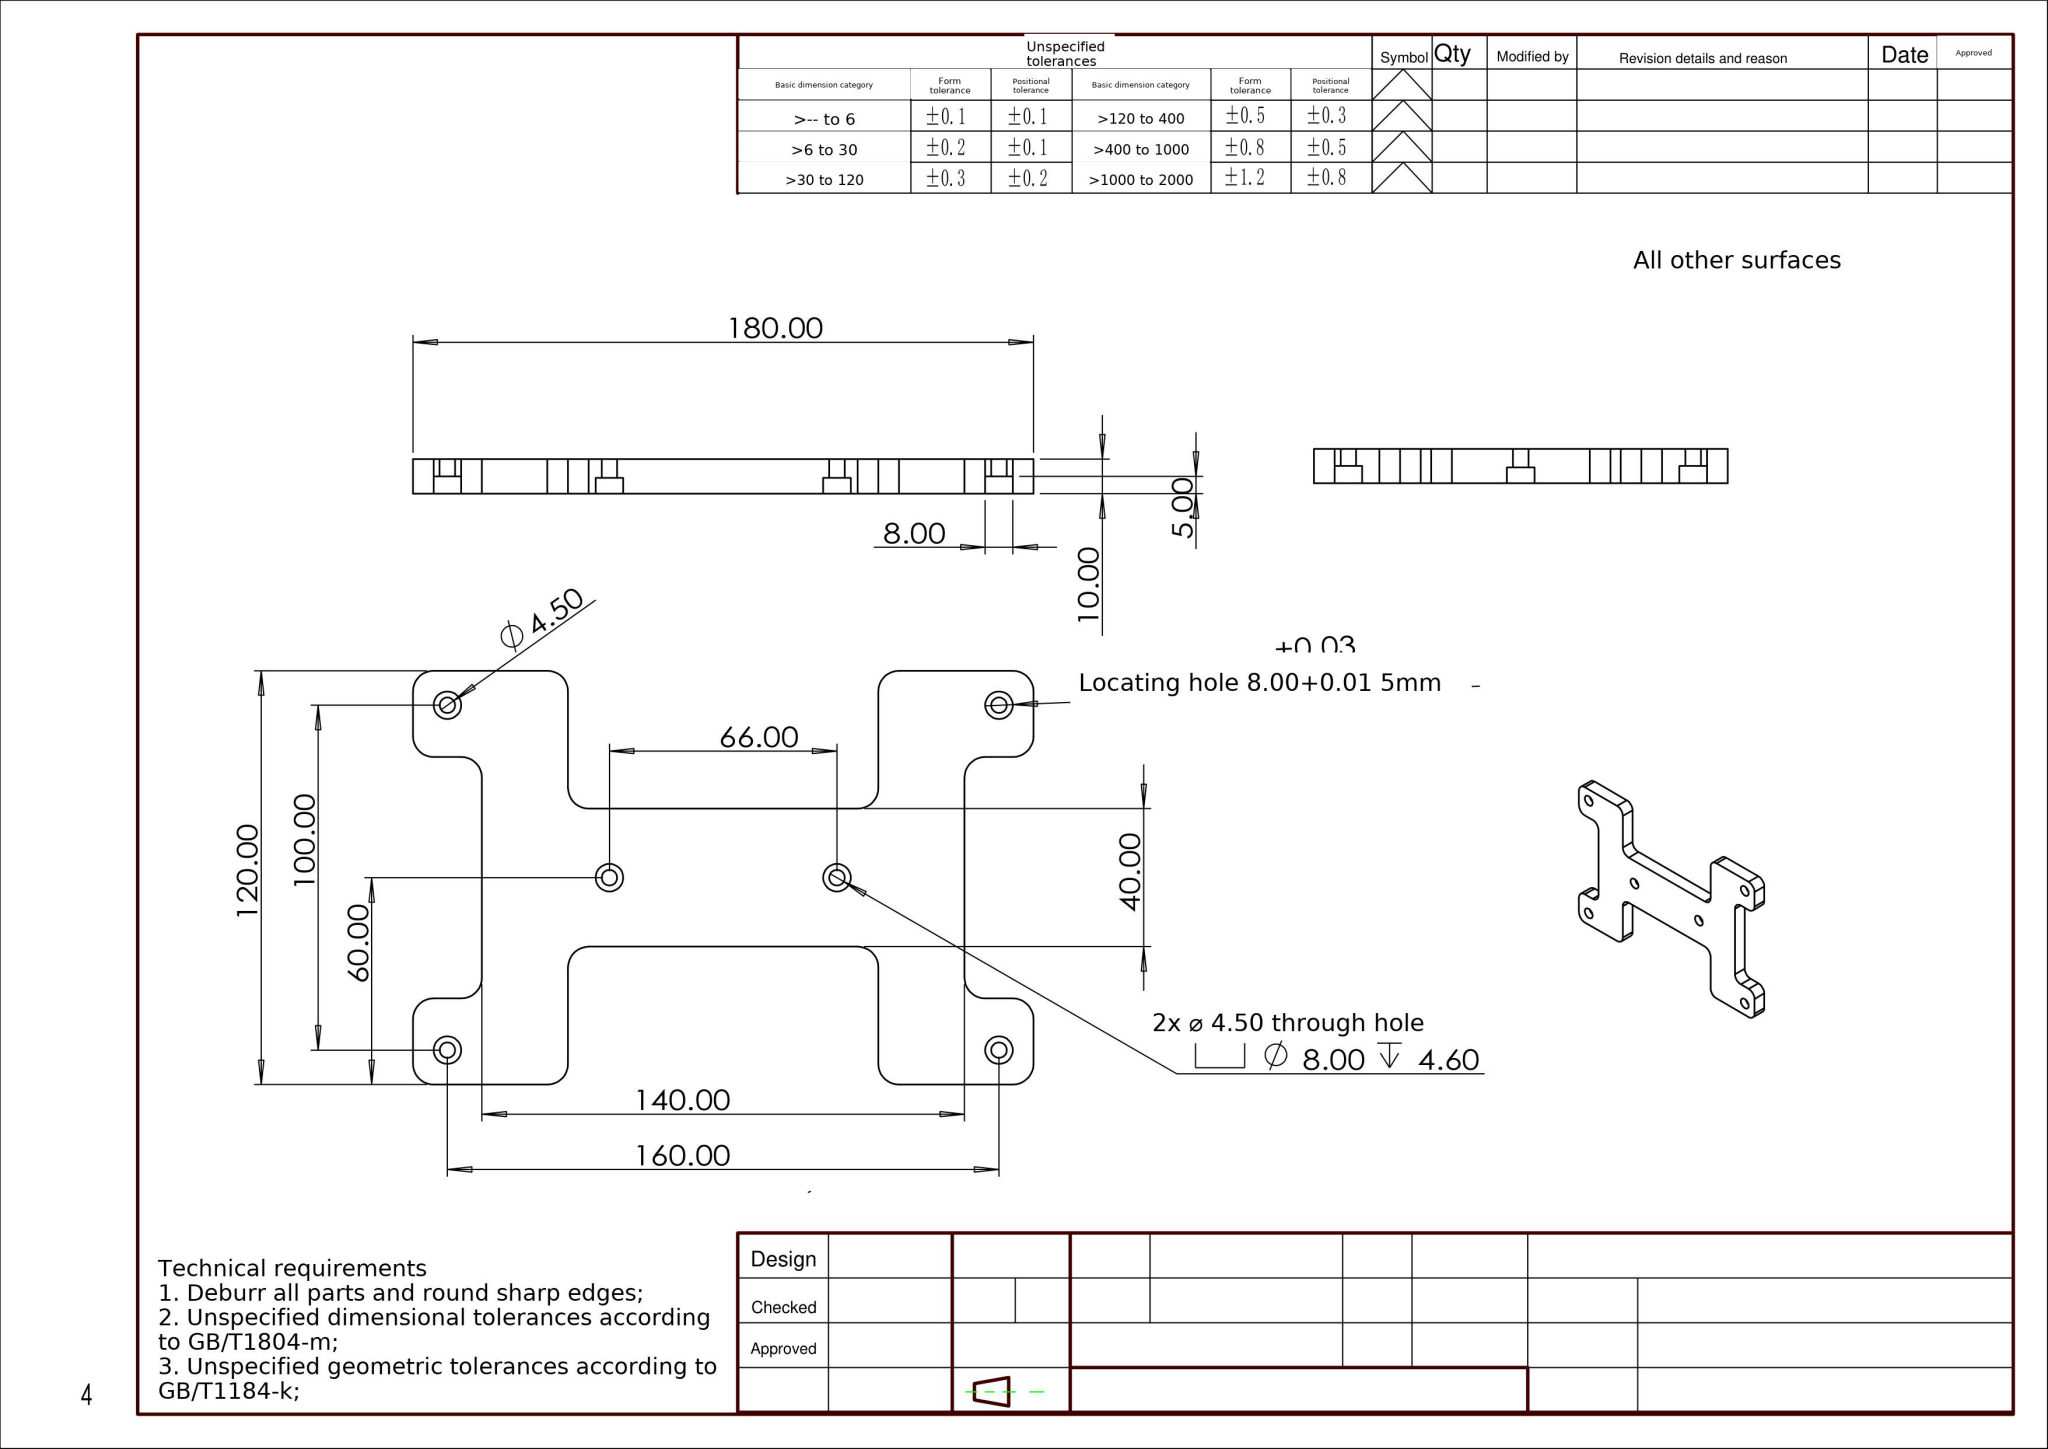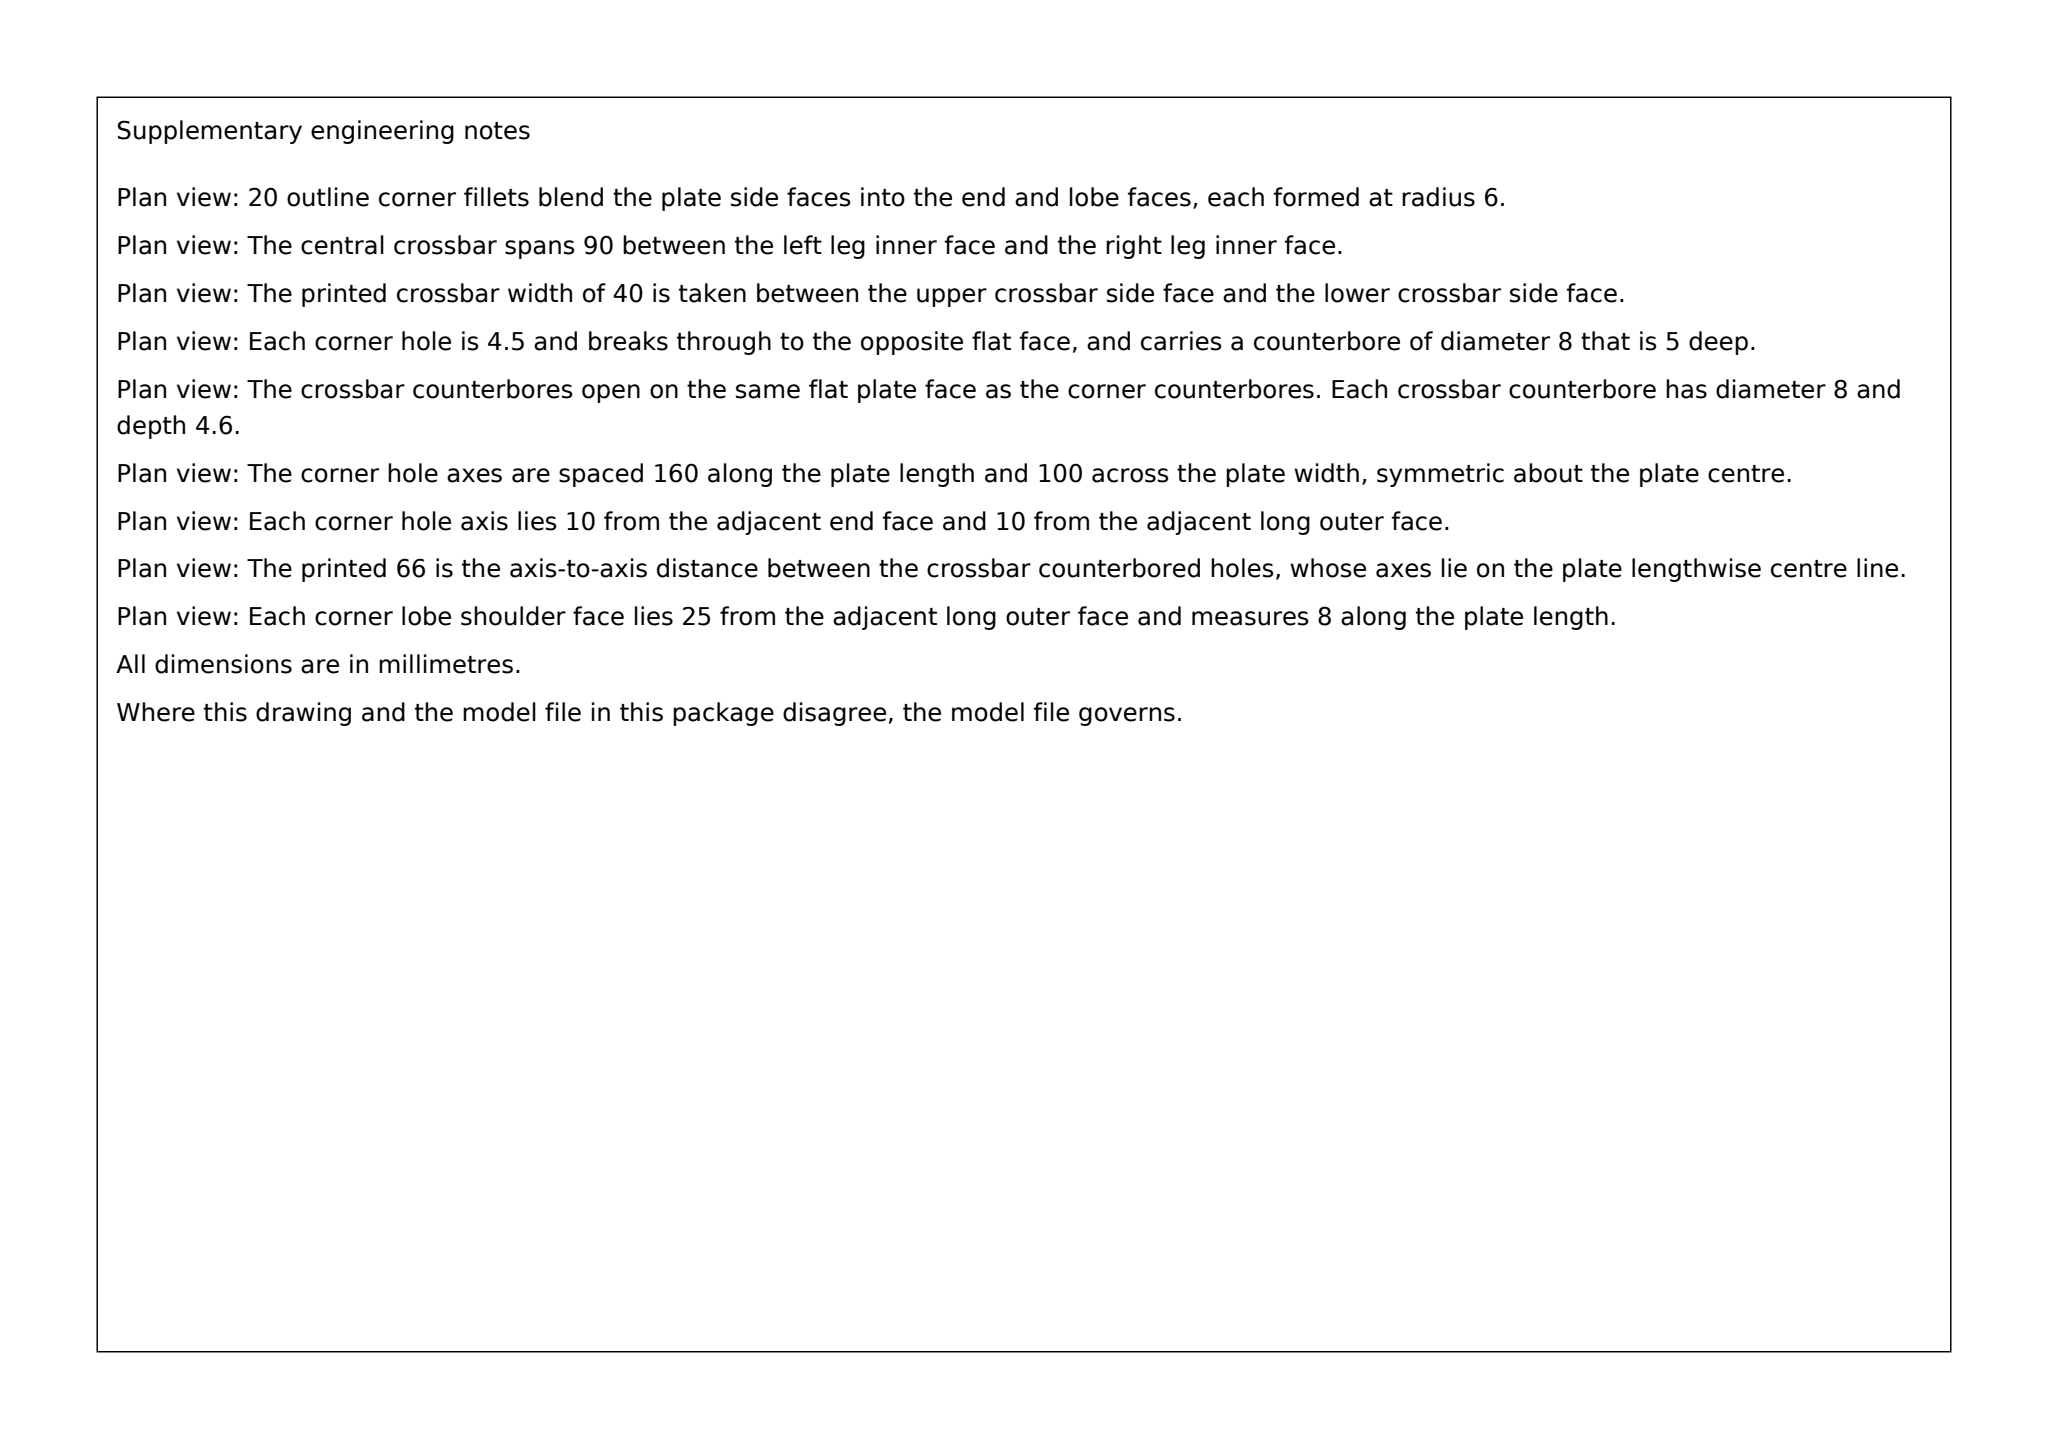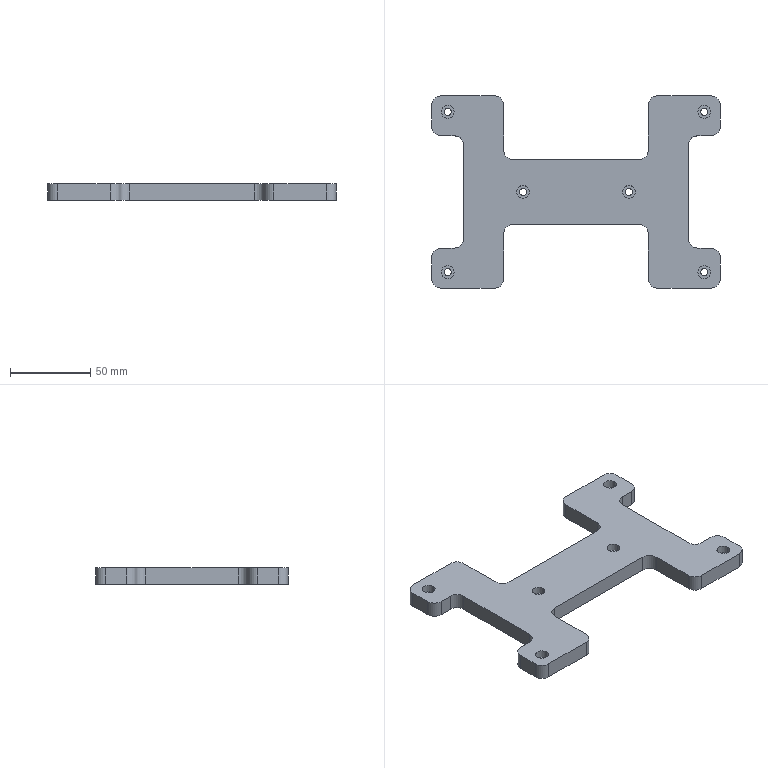Part | SolidWorks | mm | 1 solid | 72 faces | box 180 x 120 x 10 mm | volume 113733 mm3 | cylinder 44 | plane 28 | commonest cylinder face diameters 12 x20 8 x12 4.5 x12
build123d program:
from build123d import *

# Parameters (mm, degrees)
SKETCH1_W                                         = 180
SKETCH1_H                                         = 120
BOSS_EXTRUDE1_DEPTH                               = 10
SKETCH2_W                                         = 20
SKETCH2_H                                         = 70
SKETCH2_W_2                                       = 90
SKETCH2_H_2                                       = 40
CUT_EXTRUDE1_DEPTH                                = 10
SKETCH3_R                                         = 4
CUT_EXTRUDE2_DEPTH                                = 5
F_4_5_4_5_DIAMETER_HOLE1_D                        = 4.5
FILLET1_R                                         = 6
MIRROR3_COPY_1_SKETCH_R                           = 4
MIRROR3_COPY_1_DEPTH                              = 5
MIRROR3_COPY_2_D                                  = 4.5
HOLE_SIZE_ACCORDING_TO_HEXAGON_SOCKET_D           = 4.5
HOLE_SIZE_ACCORDING_TO_HEXAGON_SOCKET_CBORE_D     = 8
HOLE_SIZE_ACCORDING_TO_HEXAGON_SOCKET_CBORE_DEPTH = 4.6


with BuildPart() as part:
    # Sketch1 → Boss-Extrude1 (new body)
    with BuildSketch(Plane.XY):
        Rectangle(SKETCH1_W, SKETCH1_H)
    extrude(amount=BOSS_EXTRUDE1_DEPTH)

    # Sketch2 → Cut-Extrude1 (cut)
    with BuildSketch(Plane(origin=(0, 0, 0), x_dir=(-1, 0, 0), z_dir=(0, 0, -1))):
        with Locations((80, 0)):
            Rectangle(SKETCH2_W, SKETCH2_H)
        with Locations((0, 40)):
            Rectangle(SKETCH2_W_2, SKETCH2_H_2)
        with Locations((-80, 0)):
            Rectangle(SKETCH2_W, SKETCH2_H)
        with Locations((0, -40)):
            Rectangle(SKETCH2_W_2, SKETCH2_H_2)
    extrude(amount=-CUT_EXTRUDE1_DEPTH, mode=Mode.SUBTRACT)

    # Sketch3 → Cut-Extrude2 (cut)
    with BuildSketch(Plane.XY.offset(10)):
        with Locations((-80, 50)):
            Circle(SKETCH3_R)
    cut_extrude2 = extrude(amount=-CUT_EXTRUDE2_DEPTH, mode=Mode.SUBTRACT)

    # 4.5 _4.5_ Diameter Hole1 (through all)
    with Locations(Plane.XY.offset(5)):
        with Locations((-80, 50)):
            f_4_5_4_5_diameter_hole1 = Hole(F_4_5_4_5_DIAMETER_HOLE1_D / 2)

    # Fillet1
    fillet1_edges = [part.edges().sort_by_distance(p)[0] for p in [
        (-90, 35, 5),
        (-90, -35, 5),
        (-70, -35, 5),
        (-70, 35, 5),
        (-45, -60, 5),
        (45, -60, 5),
        (45, -20, 5),
        (-45, -20, 5),
        (70, -35, 5),
        (90, -35, 5),
        (90, 35, 5),
        (70, 35, 5),
        (-45, 60, 5),
        (-45, 20, 5),
        (45, 20, 5),
        (45, 60, 5),
        (90, -60, 5),
        (-90, -60, 5),
        (-90, 60, 5),
        (90, 60, 5),
    ]]
    fillet(fillet1_edges, radius=FILLET1_R)

    # Mirror2: Cut-Extrude2, 4.5 _4.5_ Diameter Hole1 across plane
    add(cut_extrude2.mirror(Plane(origin=(0, 0, 0), x_dir=(0, 0, 1), z_dir=(1, 0, 0))), mode=Mode.SUBTRACT)
    add(f_4_5_4_5_diameter_hole1.mirror(Plane(origin=(0, 0, 0), x_dir=(0, 0, 1), z_dir=(1, 0, 0))), mode=Mode.SUBTRACT)

    # Mirror3: Cut-Extrude2, 4.5 _4.5_ Diameter Hole1 across plane
    add(cut_extrude2.mirror(Plane.ZX), mode=Mode.SUBTRACT)
    add(f_4_5_4_5_diameter_hole1.mirror(Plane.ZX), mode=Mode.SUBTRACT)

    # Mirror3 copy 1 sketch → Mirror3 copy 1 (cut)
    with BuildSketch(Plane(origin=(0, 0, 10), x_dir=(-1, 0, 0), z_dir=(0, 0, 1))):
        with Locations((-80, 50)):
            Circle(MIRROR3_COPY_1_SKETCH_R)
    extrude(amount=-MIRROR3_COPY_1_DEPTH, mode=Mode.SUBTRACT)

    # Mirror3 copy 2 (through all)
    with Locations(Plane(origin=(0, 0, 5), x_dir=(-1, 0, 0), z_dir=(0, 0, 1))):
        with Locations((-80, 50)):
            Hole(MIRROR3_COPY_2_D / 2)

    # Hole Size _ according to_ Hexagon Socket (through all)
    with Locations(Plane.XY.offset(10)):
        with Locations((33, 0), (-33, 0)):
            CounterBoreHole(HOLE_SIZE_ACCORDING_TO_HEXAGON_SOCKET_D / 2, HOLE_SIZE_ACCORDING_TO_HEXAGON_SOCKET_CBORE_D / 2, HOLE_SIZE_ACCORDING_TO_HEXAGON_SOCKET_CBORE_DEPTH)


solid = part.part